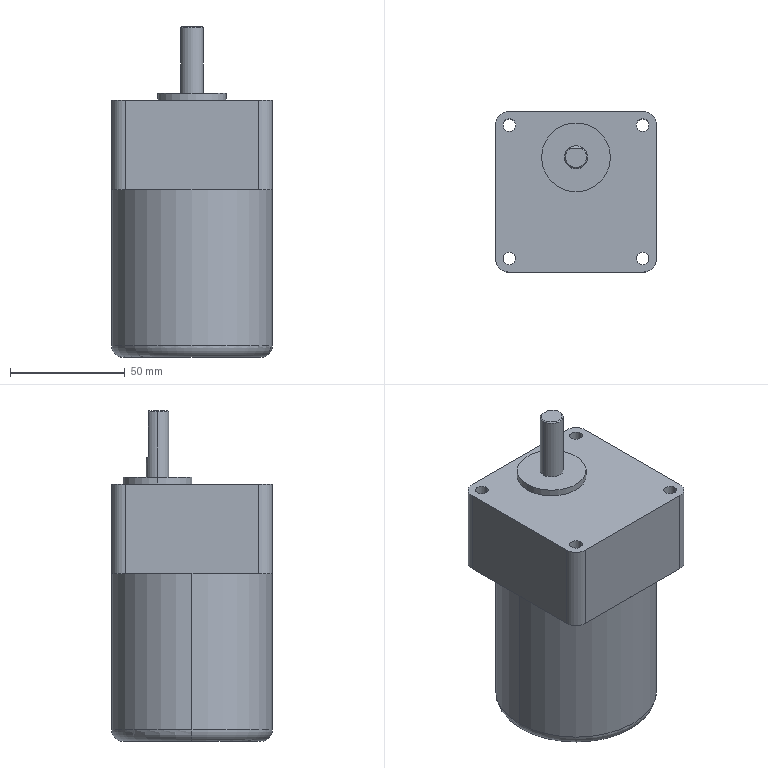Component | SolidWorks | LD101-02--Q1000-Q16-1.SLDQ1SM-1_LD101-02-3IK15Q1-C-3GN10K-1 | 1 solid | 37 faces | box 70 x 70 x 144 mm | volume 470295 mm3 | cylinder 18 | plane 14 | cone 3 | torus 2 | commonest cylinder face diameters 5.5 x8 12 x4 10 x2 30 x2 70 x2 | material SUS304
STEP:
#1=COLOUR_RGB('',0.7922,0.8196,0.9333);
#2=FILL_AREA_STYLE_COLOUR('',#1);
#3=FILL_AREA_STYLE('',(#2));
#4=SURFACE_STYLE_FILL_AREA(#3);
#5=SURFACE_SIDE_STYLE('',(#4));
#6=SURFACE_STYLE_USAGE(.BOTH.,#5);
#7=PRESENTATION_STYLE_ASSIGNMENT((#6));
#8=CARTESIAN_POINT('',(-28.624,-2.437,-4.714));
#9=VERTEX_POINT('',#8);
#10=CARTESIAN_POINT('',(-28.407,-2.437,-4.714));
#11=VERTEX_POINT('',#10);
#12=CARTESIAN_POINT('',(-28.516,-2.437,-4.714));
#13=DIRECTION('',(-0.,-0.,1.));
#14=DIRECTION('',(1.,0.,0.));
#15=AXIS2_PLACEMENT_3D('',#12,#13,#14);
#16=CIRCLE('',#15,0.1083);
#17=EDGE_CURVE('',#9,#11,#16,.T.);
#18=ORIENTED_EDGE('',*,*,#17,.F.);
#19=CARTESIAN_POINT('',(-28.624,-2.437,-3.179));
#20=VERTEX_POINT('',#19);
#21=CARTESIAN_POINT('',(-28.624,-2.437,-3.179));
#22=DIRECTION('',(-0.,-0.,1.));
#23=VECTOR('',#22,39.37);
#24=LINE('',#21,#23);
#25=EDGE_CURVE('',#9,#20,#24,.T.);
#26=ORIENTED_EDGE('',*,*,#25,.T.);
#27=CARTESIAN_POINT('',(-28.407,-2.437,-3.179));
#28=VERTEX_POINT('',#27);
#29=CARTESIAN_POINT('',(-28.516,-2.437,-3.179));
#30=DIRECTION('',(-0.,-0.,1.));
#31=DIRECTION('',(1.,0.,0.));
#32=AXIS2_PLACEMENT_3D('',#29,#30,#31);
#33=CIRCLE('',#32,0.1083);
#34=EDGE_CURVE('',#20,#28,#33,.T.);
#35=ORIENTED_EDGE('',*,*,#34,.T.);
#36=CARTESIAN_POINT('',(-28.407,-2.437,-3.179));
#37=DIRECTION('',(-0.,-0.,1.));
#38=VECTOR('',#37,39.37);
#39=LINE('',#36,#38);
#40=EDGE_CURVE('',#11,#28,#39,.T.);
#41=ORIENTED_EDGE('',*,*,#40,.F.);
#42=EDGE_LOOP('',(#18,#26,#35,#41));
#43=FACE_OUTER_BOUND('',#42,.T.);
#44=CARTESIAN_POINT('',(-28.516,-2.437,-3.179));
#45=DIRECTION('',(-0.,-0.,1.));
#46=DIRECTION('',(1.,0.,0.));
#47=AXIS2_PLACEMENT_3D('',#44,#45,#46);
#48=CYLINDRICAL_SURFACE('',#47,0.1083);
#49=ADVANCED_FACE('',(#43),#48,.F.);
#50=CARTESIAN_POINT('',(-28.624,-4.72,-4.714));
#51=VERTEX_POINT('',#50);
#52=CARTESIAN_POINT('',(-28.407,-4.72,-4.714));
#53=VERTEX_POINT('',#52);
#54=CARTESIAN_POINT('',(-28.516,-4.72,-4.714));
#55=DIRECTION('',(-0.,-0.,1.));
#56=DIRECTION('',(1.,0.,0.));
#57=AXIS2_PLACEMENT_3D('',#54,#55,#56);
#58=CIRCLE('',#57,0.1083);
#59=EDGE_CURVE('',#51,#53,#58,.T.);
#60=ORIENTED_EDGE('',*,*,#59,.F.);
#61=CARTESIAN_POINT('',(-28.624,-4.72,-3.179));
#62=VERTEX_POINT('',#61);
#63=CARTESIAN_POINT('',(-28.624,-4.72,-3.179));
#64=DIRECTION('',(-0.,-0.,1.));
#65=VECTOR('',#64,39.37);
#66=LINE('',#63,#65);
#67=EDGE_CURVE('',#51,#62,#66,.T.);
#68=ORIENTED_EDGE('',*,*,#67,.T.);
#69=CARTESIAN_POINT('',(-28.407,-4.72,-3.179));
#70=VERTEX_POINT('',#69);
#71=CARTESIAN_POINT('',(-28.516,-4.72,-3.179));
#72=DIRECTION('',(-0.,-0.,1.));
#73=DIRECTION('',(1.,0.,0.));
#74=AXIS2_PLACEMENT_3D('',#71,#72,#73);
#75=CIRCLE('',#74,0.1083);
#76=EDGE_CURVE('',#62,#70,#75,.T.);
#77=ORIENTED_EDGE('',*,*,#76,.T.);
#78=CARTESIAN_POINT('',(-28.407,-4.72,-3.179));
#79=DIRECTION('',(-0.,-0.,1.));
#80=VECTOR('',#79,39.37);
#81=LINE('',#78,#80);
#82=EDGE_CURVE('',#53,#70,#81,.T.);
#83=ORIENTED_EDGE('',*,*,#82,.F.);
#84=EDGE_LOOP('',(#60,#68,#77,#83));
#85=FACE_OUTER_BOUND('',#84,.T.);
#86=CARTESIAN_POINT('',(-28.516,-4.72,-3.179));
#87=DIRECTION('',(-0.,-0.,1.));
#88=DIRECTION('',(1.,0.,0.));
#89=AXIS2_PLACEMENT_3D('',#86,#87,#88);
#90=CYLINDRICAL_SURFACE('',#89,0.1083);
#91=ADVANCED_FACE('',(#85),#90,.F.);
#92=CARTESIAN_POINT('',(-30.907,-4.72,-4.714));
#93=VERTEX_POINT('',#92);
#94=CARTESIAN_POINT('',(-30.69,-4.72,-4.714));
#95=VERTEX_POINT('',#94);
#96=CARTESIAN_POINT('',(-30.798,-4.72,-4.714));
#97=DIRECTION('',(-0.,-0.,1.));
#98=DIRECTION('',(1.,0.,0.));
#99=AXIS2_PLACEMENT_3D('',#96,#97,#98);
#100=CIRCLE('',#99,0.1083);
#101=EDGE_CURVE('',#93,#95,#100,.T.);
#102=ORIENTED_EDGE('',*,*,#101,.F.);
#103=CARTESIAN_POINT('',(-30.907,-4.72,-3.179));
#104=VERTEX_POINT('',#103);
#105=CARTESIAN_POINT('',(-30.907,-4.72,-3.179));
#106=DIRECTION('',(-0.,-0.,1.));
#107=VECTOR('',#106,39.37);
#108=LINE('',#105,#107);
#109=EDGE_CURVE('',#93,#104,#108,.T.);
#110=ORIENTED_EDGE('',*,*,#109,.T.);
#111=CARTESIAN_POINT('',(-30.69,-4.72,-3.179));
#112=VERTEX_POINT('',#111);
#113=CARTESIAN_POINT('',(-30.798,-4.72,-3.179));
#114=DIRECTION('',(-0.,-0.,1.));
#115=DIRECTION('',(1.,0.,0.));
#116=AXIS2_PLACEMENT_3D('',#113,#114,#115);
#117=CIRCLE('',#116,0.1083);
#118=EDGE_CURVE('',#104,#112,#117,.T.);
#119=ORIENTED_EDGE('',*,*,#118,.T.);
#120=CARTESIAN_POINT('',(-30.69,-4.72,-3.179));
#121=DIRECTION('',(-0.,-0.,1.));
#122=VECTOR('',#121,39.37);
#123=LINE('',#120,#122);
#124=EDGE_CURVE('',#95,#112,#123,.T.);
#125=ORIENTED_EDGE('',*,*,#124,.F.);
#126=EDGE_LOOP('',(#102,#110,#119,#125));
#127=FACE_OUTER_BOUND('',#126,.T.);
#128=CARTESIAN_POINT('',(-30.798,-4.72,-3.179));
#129=DIRECTION('',(-0.,-0.,1.));
#130=DIRECTION('',(1.,0.,0.));
#131=AXIS2_PLACEMENT_3D('',#128,#129,#130);
#132=CYLINDRICAL_SURFACE('',#131,0.1083);
#133=ADVANCED_FACE('',(#127),#132,.F.);
#134=CARTESIAN_POINT('',(-30.907,-2.437,-4.714));
#135=VERTEX_POINT('',#134);
#136=CARTESIAN_POINT('',(-30.69,-2.437,-4.714));
#137=VERTEX_POINT('',#136);
#138=CARTESIAN_POINT('',(-30.798,-2.437,-4.714));
#139=DIRECTION('',(-0.,-0.,1.));
#140=DIRECTION('',(1.,0.,0.));
#141=AXIS2_PLACEMENT_3D('',#138,#139,#140);
#142=CIRCLE('',#141,0.1083);
#143=EDGE_CURVE('',#135,#137,#142,.T.);
#144=ORIENTED_EDGE('',*,*,#143,.F.);
#145=CARTESIAN_POINT('',(-30.907,-2.437,-3.179));
#146=VERTEX_POINT('',#145);
#147=CARTESIAN_POINT('',(-30.907,-2.437,-3.179));
#148=DIRECTION('',(-0.,-0.,1.));
#149=VECTOR('',#148,39.37);
#150=LINE('',#147,#149);
#151=EDGE_CURVE('',#135,#146,#150,.T.);
#152=ORIENTED_EDGE('',*,*,#151,.T.);
#153=CARTESIAN_POINT('',(-30.69,-2.437,-3.179));
#154=VERTEX_POINT('',#153);
#155=CARTESIAN_POINT('',(-30.798,-2.437,-3.179));
#156=DIRECTION('',(-0.,-0.,1.));
#157=DIRECTION('',(1.,0.,0.));
#158=AXIS2_PLACEMENT_3D('',#155,#156,#157);
#159=CIRCLE('',#158,0.1083);
#160=EDGE_CURVE('',#146,#154,#159,.T.);
#161=ORIENTED_EDGE('',*,*,#160,.T.);
#162=CARTESIAN_POINT('',(-30.69,-2.437,-3.179));
#163=DIRECTION('',(-0.,-0.,1.));
#164=VECTOR('',#163,39.37);
#165=LINE('',#162,#164);
#166=EDGE_CURVE('',#137,#154,#165,.T.);
#167=ORIENTED_EDGE('',*,*,#166,.F.);
#168=EDGE_LOOP('',(#144,#152,#161,#167));
#169=FACE_OUTER_BOUND('',#168,.T.);
#170=CARTESIAN_POINT('',(-30.798,-2.437,-3.179));
#171=DIRECTION('',(-0.,-0.,1.));
#172=DIRECTION('',(1.,0.,0.));
#173=AXIS2_PLACEMENT_3D('',#170,#171,#172);
#174=CYLINDRICAL_SURFACE('',#173,0.1083);
#175=ADVANCED_FACE('',(#169),#174,.F.);
#176=CARTESIAN_POINT('',(-29.48,-2.988,-1.919));
#177=VERTEX_POINT('',#176);
#178=CARTESIAN_POINT('',(-29.576,-2.831,-1.919));
#179=VERTEX_POINT('',#178);
#180=CARTESIAN_POINT('',(-29.657,-2.988,-1.919));
#181=DIRECTION('',(-0.,-0.,1.));
#182=DIRECTION('',(1.,0.,0.));
#183=AXIS2_PLACEMENT_3D('',#180,#181,#182);
#184=CIRCLE('',#183,0.1772);
#185=EDGE_CURVE('',#177,#179,#184,.T.);
#186=ORIENTED_EDGE('',*,*,#185,.F.);
#187=CARTESIAN_POINT('',(-29.46,-2.988,-1.939));
#188=VERTEX_POINT('',#187);
#189=CARTESIAN_POINT('',(-29.48,-2.988,-1.919));
#190=DIRECTION('',(0.7071,0.,-0.7071));
#191=VECTOR('',#190,39.37);
#192=LINE('',#189,#191);
#193=EDGE_CURVE('',#177,#188,#192,.T.);
#194=ORIENTED_EDGE('',*,*,#193,.T.);
#195=CARTESIAN_POINT('',(-29.539,-2.831,-1.939));
#196=VERTEX_POINT('',#195);
#197=CARTESIAN_POINT('',(-29.657,-2.988,-1.939));
#198=DIRECTION('',(0.,0.,-1.));
#199=DIRECTION('',(1.,0.,0.));
#200=AXIS2_PLACEMENT_3D('',#197,#198,#199);
#201=CIRCLE('',#200,0.1969);
#202=EDGE_CURVE('',#196,#188,#201,.T.);
#203=ORIENTED_EDGE('',*,*,#202,.F.);
#204=CARTESIAN_POINT('',(-29.576,-2.831,-1.919));
#205=CARTESIAN_POINT('',(-29.563,-2.831,-1.925));
#206=CARTESIAN_POINT('',(-29.551,-2.831,-1.932));
#207=CARTESIAN_POINT('',(-29.539,-2.831,-1.939));
#208=B_SPLINE_CURVE_WITH_KNOTS('',3,(#204,#205,#206,#207),.UNSPECIFIED.,.F.,.F.,(4,4),(0.01478,0.01585),.UNSPECIFIED.);
#209=EDGE_CURVE('',#179,#196,#208,.T.);
#210=ORIENTED_EDGE('',*,*,#209,.F.);
#211=EDGE_LOOP('',(#186,#194,#203,#210));
#212=FACE_OUTER_BOUND('',#211,.T.);
#213=CARTESIAN_POINT('',(-29.657,-2.988,-1.919));
#214=DIRECTION('',(0.,0.,-1.));
#215=DIRECTION('',(-1.,0.,0.));
#216=AXIS2_PLACEMENT_3D('',#213,#214,#215);
#217=CONICAL_SURFACE('',#216,0.1772,0.7854);
#218=ADVANCED_FACE('',(#212),#217,.T.);
#219=ORIENTED_EDGE('',*,*,#193,.F.);
#220=CARTESIAN_POINT('',(-29.834,-2.988,-1.919));
#221=VERTEX_POINT('',#220);
#222=CARTESIAN_POINT('',(-29.657,-2.988,-1.919));
#223=DIRECTION('',(-0.,-0.,1.));
#224=DIRECTION('',(1.,0.,0.));
#225=AXIS2_PLACEMENT_3D('',#222,#223,#224);
#226=CIRCLE('',#225,0.1772);
#227=EDGE_CURVE('',#221,#177,#226,.T.);
#228=ORIENTED_EDGE('',*,*,#227,.F.);
#229=CARTESIAN_POINT('',(-29.854,-2.988,-1.939));
#230=VERTEX_POINT('',#229);
#231=CARTESIAN_POINT('',(-29.834,-2.988,-1.919));
#232=DIRECTION('',(-0.7071,0.,-0.7071));
#233=VECTOR('',#232,39.37);
#234=LINE('',#231,#233);
#235=EDGE_CURVE('',#221,#230,#234,.T.);
#236=ORIENTED_EDGE('',*,*,#235,.T.);
#237=CARTESIAN_POINT('',(-29.657,-2.988,-1.939));
#238=DIRECTION('',(0.,0.,-1.));
#239=DIRECTION('',(1.,0.,0.));
#240=AXIS2_PLACEMENT_3D('',#237,#238,#239);
#241=CIRCLE('',#240,0.1969);
#242=EDGE_CURVE('',#188,#230,#241,.T.);
#243=ORIENTED_EDGE('',*,*,#242,.F.);
#244=EDGE_LOOP('',(#219,#228,#236,#243));
#245=FACE_OUTER_BOUND('',#244,.T.);
#246=CARTESIAN_POINT('',(-29.657,-2.988,-1.919));
#247=DIRECTION('',(0.,0.,-1.));
#248=DIRECTION('',(-1.,0.,0.));
#249=AXIS2_PLACEMENT_3D('',#246,#247,#248);
#250=CONICAL_SURFACE('',#249,0.1772,0.7854);
#251=ADVANCED_FACE('',(#245),#250,.T.);
#252=ORIENTED_EDGE('',*,*,#202,.T.);
#253=CARTESIAN_POINT('',(-29.46,-2.988,-3.061));
#254=VERTEX_POINT('',#253);
#255=CARTESIAN_POINT('',(-29.46,-2.988,-1.919));
#256=DIRECTION('',(0.,0.,-1.));
#257=VECTOR('',#256,39.37);
#258=LINE('',#255,#257);
#259=EDGE_CURVE('',#188,#254,#258,.T.);
#260=ORIENTED_EDGE('',*,*,#259,.T.);
#261=CARTESIAN_POINT('',(-29.854,-2.988,-3.061));
#262=VERTEX_POINT('',#261);
#263=CARTESIAN_POINT('',(-29.657,-2.988,-3.061));
#264=DIRECTION('',(0.,0.,-1.));
#265=DIRECTION('',(1.,0.,0.));
#266=AXIS2_PLACEMENT_3D('',#263,#264,#265);
#267=CIRCLE('',#266,0.1969);
#268=EDGE_CURVE('',#262,#254,#267,.T.);
#269=ORIENTED_EDGE('',*,*,#268,.F.);
#270=CARTESIAN_POINT('',(-29.854,-2.988,-1.919));
#271=DIRECTION('',(0.,0.,-1.));
#272=VECTOR('',#271,39.37);
#273=LINE('',#270,#272);
#274=EDGE_CURVE('',#230,#262,#273,.T.);
#275=ORIENTED_EDGE('',*,*,#274,.F.);
#276=CARTESIAN_POINT('',(-29.775,-2.831,-1.939));
#277=VERTEX_POINT('',#276);
#278=CARTESIAN_POINT('',(-29.657,-2.988,-1.939));
#279=DIRECTION('',(0.,0.,-1.));
#280=DIRECTION('',(1.,-0.,0.));
#281=AXIS2_PLACEMENT_3D('',#278,#279,#280);
#282=CIRCLE('',#281,0.1969);
#283=EDGE_CURVE('',#230,#277,#282,.T.);
#284=ORIENTED_EDGE('',*,*,#283,.T.);
#285=CARTESIAN_POINT('',(-29.775,-2.831,-2.706));
#286=VERTEX_POINT('',#285);
#287=CARTESIAN_POINT('',(-29.775,-2.831,-1.919));
#288=DIRECTION('',(0.,0.,-1.));
#289=VECTOR('',#288,39.37);
#290=LINE('',#287,#289);
#291=EDGE_CURVE('',#277,#286,#290,.T.);
#292=ORIENTED_EDGE('',*,*,#291,.T.);
#293=CARTESIAN_POINT('',(-29.539,-2.831,-2.706));
#294=VERTEX_POINT('',#293);
#295=CARTESIAN_POINT('',(-29.775,-2.831,-2.706));
#296=CARTESIAN_POINT('',(-29.703,-2.776,-2.761));
#297=CARTESIAN_POINT('',(-29.612,-2.776,-2.761));
#298=CARTESIAN_POINT('',(-29.539,-2.831,-2.706));
#299=(BOUNDED_CURVE()B_SPLINE_CURVE(3,(#295,#296,#297,#298),.UNSPECIFIED.,.F.,.F.)B_SPLINE_CURVE_WITH_KNOTS((4,4),(5.64,6.927),.UNSPECIFIED.)CURVE()GEOMETRIC_REPRESENTATION_ITEM()RATIONAL_B_SPLINE_CURVE((1.,0.8667,0.8667,1.))REPRESENTATION_ITEM(''));
#300=EDGE_CURVE('',#286,#294,#299,.T.);
#301=ORIENTED_EDGE('',*,*,#300,.T.);
#302=CARTESIAN_POINT('',(-29.539,-2.831,-1.919));
#303=DIRECTION('',(-0.,-0.,1.));
#304=VECTOR('',#303,39.37);
#305=LINE('',#302,#304);
#306=EDGE_CURVE('',#294,#196,#305,.T.);
#307=ORIENTED_EDGE('',*,*,#306,.T.);
#308=EDGE_LOOP('',(#252,#260,#269,#275,#284,#292,#301,#307));
#309=FACE_OUTER_BOUND('',#308,.T.);
#310=CARTESIAN_POINT('',(-29.657,-2.988,-1.919));
#311=DIRECTION('',(0.,0.,-1.));
#312=DIRECTION('',(-1.,0.,0.));
#313=AXIS2_PLACEMENT_3D('',#310,#311,#312);
#314=CYLINDRICAL_SURFACE('',#313,0.1969);
#315=ADVANCED_FACE('',(#309),#314,.T.);
#316=CARTESIAN_POINT('',(-29.067,-2.988,-3.061));
#317=VERTEX_POINT('',#316);
#318=CARTESIAN_POINT('',(-30.248,-2.988,-3.061));
#319=VERTEX_POINT('',#318);
#320=CARTESIAN_POINT('',(-29.657,-2.988,-3.061));
#321=DIRECTION('',(-0.,-0.,1.));
#322=DIRECTION('',(1.,0.,0.));
#323=AXIS2_PLACEMENT_3D('',#320,#321,#322);
#324=CIRCLE('',#323,0.5906);
#325=EDGE_CURVE('',#317,#319,#324,.T.);
#326=ORIENTED_EDGE('',*,*,#325,.F.);
#327=CARTESIAN_POINT('',(-29.067,-2.988,-3.179));
#328=VERTEX_POINT('',#327);
#329=CARTESIAN_POINT('',(-29.067,-2.988,-3.061));
#330=DIRECTION('',(0.,0.,-1.));
#331=VECTOR('',#330,39.37);
#332=LINE('',#329,#331);
#333=EDGE_CURVE('',#317,#328,#332,.T.);
#334=ORIENTED_EDGE('',*,*,#333,.T.);
#335=CARTESIAN_POINT('',(-30.248,-2.988,-3.179));
#336=VERTEX_POINT('',#335);
#337=CARTESIAN_POINT('',(-29.657,-2.988,-3.179));
#338=DIRECTION('',(-0.,-0.,1.));
#339=DIRECTION('',(1.,0.,0.));
#340=AXIS2_PLACEMENT_3D('',#337,#338,#339);
#341=CIRCLE('',#340,0.5906);
#342=EDGE_CURVE('',#328,#336,#341,.T.);
#343=ORIENTED_EDGE('',*,*,#342,.T.);
#344=CARTESIAN_POINT('',(-30.248,-2.988,-3.061));
#345=DIRECTION('',(0.,0.,-1.));
#346=VECTOR('',#345,39.37);
#347=LINE('',#344,#346);
#348=EDGE_CURVE('',#319,#336,#347,.T.);
#349=ORIENTED_EDGE('',*,*,#348,.F.);
#350=EDGE_LOOP('',(#326,#334,#343,#349));
#351=FACE_OUTER_BOUND('',#350,.T.);
#352=CARTESIAN_POINT('',(-29.657,-2.988,-3.061));
#353=DIRECTION('',(0.,0.,-1.));
#354=DIRECTION('',(-1.,0.,-0.));
#355=AXIS2_PLACEMENT_3D('',#352,#353,#354);
#356=CYLINDRICAL_SURFACE('',#355,0.5906);
#357=ADVANCED_FACE('',(#351),#356,.T.);
#358=CARTESIAN_POINT('',(-30.838,-3.579,-7.588));
#359=VERTEX_POINT('',#358);
#360=CARTESIAN_POINT('',(-28.476,-3.579,-7.588));
#361=VERTEX_POINT('',#360);
#362=CARTESIAN_POINT('',(-29.657,-3.579,-7.588));
#363=DIRECTION('',(0.,0.,-1.));
#364=DIRECTION('',(1.,0.,0.));
#365=AXIS2_PLACEMENT_3D('',#362,#363,#364);
#366=CIRCLE('',#365,1.181);
#367=EDGE_CURVE('',#359,#361,#366,.T.);
#368=ORIENTED_EDGE('',*,*,#367,.F.);
#369=CARTESIAN_POINT('',(-31.035,-3.579,-7.391));
#370=VERTEX_POINT('',#369);
#371=CARTESIAN_POINT('',(-30.838,-3.579,-7.391));
#372=DIRECTION('',(0.,1.,0.));
#373=DIRECTION('',(-1.,0.,0.));
#374=AXIS2_PLACEMENT_3D('',#371,#372,#373);
#375=CIRCLE('',#374,0.1969);
#376=EDGE_CURVE('',#359,#370,#375,.T.);
#377=ORIENTED_EDGE('',*,*,#376,.T.);
#378=CARTESIAN_POINT('',(-28.279,-3.579,-7.391));
#379=VERTEX_POINT('',#378);
#380=CARTESIAN_POINT('',(-29.657,-3.579,-7.391));
#381=DIRECTION('',(-0.,-0.,1.));
#382=DIRECTION('',(1.,0.,0.));
#383=AXIS2_PLACEMENT_3D('',#380,#381,#382);
#384=CIRCLE('',#383,1.378);
#385=EDGE_CURVE('',#379,#370,#384,.T.);
#386=ORIENTED_EDGE('',*,*,#385,.F.);
#387=CARTESIAN_POINT('',(-28.476,-3.579,-7.391));
#388=DIRECTION('',(-0.,-1.,-0.));
#389=DIRECTION('',(1.,0.,0.));
#390=AXIS2_PLACEMENT_3D('',#387,#388,#389);
#391=CIRCLE('',#390,0.1969);
#392=EDGE_CURVE('',#361,#379,#391,.T.);
#393=ORIENTED_EDGE('',*,*,#392,.F.);
#394=EDGE_LOOP('',(#368,#377,#386,#393));
#395=FACE_OUTER_BOUND('',#394,.T.);
#396=CARTESIAN_POINT('',(-29.657,-3.579,-7.391));
#397=DIRECTION('',(-0.,-0.,1.));
#398=DIRECTION('',(1.,0.,0.));
#399=AXIS2_PLACEMENT_3D('',#396,#397,#398);
#400=TOROIDAL_SURFACE('',#399,1.181,0.1969);
#401=ADVANCED_FACE('',(#395),#400,.T.);
#402=ORIENTED_EDGE('',*,*,#385,.T.);
#403=CARTESIAN_POINT('',(-31.035,-3.579,-4.714));
#404=VERTEX_POINT('',#403);
#405=CARTESIAN_POINT('',(-31.035,-3.579,-7.588));
#406=DIRECTION('',(-0.,-0.,1.));
#407=VECTOR('',#406,39.37);
#408=LINE('',#405,#407);
#409=EDGE_CURVE('',#370,#404,#408,.T.);
#410=ORIENTED_EDGE('',*,*,#409,.T.);
#411=CARTESIAN_POINT('',(-29.657,-2.201,-4.714));
#412=VERTEX_POINT('',#411);
#413=CARTESIAN_POINT('',(-29.657,-3.579,-4.714));
#414=DIRECTION('',(-0.,-0.,1.));
#415=DIRECTION('',(1.,0.,0.));
#416=AXIS2_PLACEMENT_3D('',#413,#414,#415);
#417=CIRCLE('',#416,1.378);
#418=EDGE_CURVE('',#412,#404,#417,.T.);
#419=ORIENTED_EDGE('',*,*,#418,.F.);
#420=CARTESIAN_POINT('',(-28.279,-3.579,-4.714));
#421=VERTEX_POINT('',#420);
#422=CARTESIAN_POINT('',(-29.657,-3.579,-4.714));
#423=DIRECTION('',(-0.,-0.,1.));
#424=DIRECTION('',(1.,0.,0.));
#425=AXIS2_PLACEMENT_3D('',#422,#423,#424);
#426=CIRCLE('',#425,1.378);
#427=EDGE_CURVE('',#421,#412,#426,.T.);
#428=ORIENTED_EDGE('',*,*,#427,.F.);
#429=CARTESIAN_POINT('',(-28.279,-3.579,-7.588));
#430=DIRECTION('',(-0.,-0.,1.));
#431=VECTOR('',#430,39.37);
#432=LINE('',#429,#431);
#433=EDGE_CURVE('',#379,#421,#432,.T.);
#434=ORIENTED_EDGE('',*,*,#433,.F.);
#435=EDGE_LOOP('',(#402,#410,#419,#428,#434));
#436=FACE_OUTER_BOUND('',#435,.T.);
#437=CARTESIAN_POINT('',(-29.657,-3.579,-7.588));
#438=DIRECTION('',(-0.,-0.,1.));
#439=DIRECTION('',(1.,0.,0.));
#440=AXIS2_PLACEMENT_3D('',#437,#438,#439);
#441=CYLINDRICAL_SURFACE('',#440,1.378);
#442=ADVANCED_FACE('',(#436),#441,.T.);
#443=CARTESIAN_POINT('',(-29.657,-2.988,-3.061));
#444=DIRECTION('',(-0.,-0.,1.));
#445=DIRECTION('',(1.,0.,0.));
#446=AXIS2_PLACEMENT_3D('',#443,#444,#445);
#447=CIRCLE('',#446,0.5906);
#448=EDGE_CURVE('',#319,#317,#447,.T.);
#449=ORIENTED_EDGE('',*,*,#448,.T.);
#450=ORIENTED_EDGE('',*,*,#325,.T.);
#451=EDGE_LOOP('',(#449,#450));
#452=FACE_OUTER_BOUND('',#451,.T.);
#453=ORIENTED_EDGE('',*,*,#268,.T.);
#454=CARTESIAN_POINT('',(-29.657,-2.988,-3.061));
#455=DIRECTION('',(0.,0.,-1.));
#456=DIRECTION('',(1.,0.,0.));
#457=AXIS2_PLACEMENT_3D('',#454,#455,#456);
#458=CIRCLE('',#457,0.1969);
#459=EDGE_CURVE('',#254,#262,#458,.T.);
#460=ORIENTED_EDGE('',*,*,#459,.T.);
#461=EDGE_LOOP('',(#453,#460));
#462=FACE_BOUND('',#461,.T.);
#463=CARTESIAN_POINT('',(-29.657,-2.988,-3.061));
#464=DIRECTION('',(-0.,-0.,1.));
#465=DIRECTION('',(1.,-0.,0.));
#466=AXIS2_PLACEMENT_3D('',#463,#464,#465);
#467=PLANE('',#466);
#468=ADVANCED_FACE('',(#452,#462),#467,.T.);
#469=CARTESIAN_POINT('',(-28.516,-2.437,-3.179));
#470=DIRECTION('',(-0.,-0.,1.));
#471=DIRECTION('',(1.,0.,0.));
#472=AXIS2_PLACEMENT_3D('',#469,#470,#471);
#473=CIRCLE('',#472,0.1083);
#474=EDGE_CURVE('',#28,#20,#473,.T.);
#475=ORIENTED_EDGE('',*,*,#474,.F.);
#476=ORIENTED_EDGE('',*,*,#34,.F.);
#477=EDGE_LOOP('',(#475,#476));
#478=FACE_BOUND('',#477,.T.);
#479=CARTESIAN_POINT('',(-28.516,-4.72,-3.179));
#480=DIRECTION('',(-0.,-0.,1.));
#481=DIRECTION('',(1.,0.,0.));
#482=AXIS2_PLACEMENT_3D('',#479,#480,#481);
#483=CIRCLE('',#482,0.1083);
#484=EDGE_CURVE('',#70,#62,#483,.T.);
#485=ORIENTED_EDGE('',*,*,#484,.F.);
#486=ORIENTED_EDGE('',*,*,#76,.F.);
#487=EDGE_LOOP('',(#485,#486));
#488=FACE_BOUND('',#487,.T.);
#489=CARTESIAN_POINT('',(-30.798,-4.72,-3.179));
#490=DIRECTION('',(-0.,-0.,1.));
#491=DIRECTION('',(1.,0.,0.));
#492=AXIS2_PLACEMENT_3D('',#489,#490,#491);
#493=CIRCLE('',#492,0.1083);
#494=EDGE_CURVE('',#112,#104,#493,.T.);
#495=ORIENTED_EDGE('',*,*,#494,.F.);
#496=ORIENTED_EDGE('',*,*,#118,.F.);
#497=EDGE_LOOP('',(#495,#496));
#498=FACE_BOUND('',#497,.T.);
#499=CARTESIAN_POINT('',(-30.798,-2.437,-3.179));
#500=DIRECTION('',(-0.,-0.,1.));
#501=DIRECTION('',(1.,0.,0.));
#502=AXIS2_PLACEMENT_3D('',#499,#500,#501);
#503=CIRCLE('',#502,0.1083);
#504=EDGE_CURVE('',#154,#146,#503,.T.);
#505=ORIENTED_EDGE('',*,*,#504,.F.);
#506=ORIENTED_EDGE('',*,*,#160,.F.);
#507=EDGE_LOOP('',(#505,#506));
#508=FACE_BOUND('',#507,.T.);
#509=CARTESIAN_POINT('',(-28.515,-4.957,-3.179));
#510=VERTEX_POINT('',#509);
#511=CARTESIAN_POINT('',(-28.279,-4.72,-3.179));
#512=VERTEX_POINT('',#511);
#513=CARTESIAN_POINT('',(-28.515,-4.72,-3.179));
#514=DIRECTION('',(-0.,-0.,1.));
#515=DIRECTION('',(1.,0.,0.));
#516=AXIS2_PLACEMENT_3D('',#513,#514,#515);
#517=CIRCLE('',#516,0.2362);
#518=EDGE_CURVE('',#510,#512,#517,.T.);
#519=ORIENTED_EDGE('',*,*,#518,.T.);
#520=CARTESIAN_POINT('',(-28.279,-2.437,-3.179));
#521=VERTEX_POINT('',#520);
#522=CARTESIAN_POINT('',(-28.279,-4.72,-3.179));
#523=DIRECTION('',(-0.,1.,0.));
#524=VECTOR('',#523,39.37);
#525=LINE('',#522,#524);
#526=EDGE_CURVE('',#512,#521,#525,.T.);
#527=ORIENTED_EDGE('',*,*,#526,.T.);
#528=CARTESIAN_POINT('',(-28.515,-2.201,-3.179));
#529=VERTEX_POINT('',#528);
#530=CARTESIAN_POINT('',(-28.515,-2.437,-3.179));
#531=DIRECTION('',(-0.,-0.,1.));
#532=DIRECTION('',(1.,0.,0.));
#533=AXIS2_PLACEMENT_3D('',#530,#531,#532);
#534=CIRCLE('',#533,0.2362);
#535=EDGE_CURVE('',#521,#529,#534,.T.);
#536=ORIENTED_EDGE('',*,*,#535,.T.);
#537=CARTESIAN_POINT('',(-30.799,-2.201,-3.179));
#538=VERTEX_POINT('',#537);
#539=CARTESIAN_POINT('',(-28.515,-2.201,-3.179));
#540=DIRECTION('',(-1.,0.,-0.));
#541=VECTOR('',#540,39.37);
#542=LINE('',#539,#541);
#543=EDGE_CURVE('',#529,#538,#542,.T.);
#544=ORIENTED_EDGE('',*,*,#543,.T.);
#545=CARTESIAN_POINT('',(-31.035,-2.437,-3.179));
#546=VERTEX_POINT('',#545);
#547=CARTESIAN_POINT('',(-30.799,-2.437,-3.179));
#548=DIRECTION('',(-0.,-0.,1.));
#549=DIRECTION('',(1.,0.,0.));
#550=AXIS2_PLACEMENT_3D('',#547,#548,#549);
#551=CIRCLE('',#550,0.2362);
#552=EDGE_CURVE('',#538,#546,#551,.T.);
#553=ORIENTED_EDGE('',*,*,#552,.T.);
#554=CARTESIAN_POINT('',(-31.035,-4.72,-3.179));
#555=VERTEX_POINT('',#554);
#556=CARTESIAN_POINT('',(-31.035,-2.437,-3.179));
#557=DIRECTION('',(-0.,-1.,-0.));
#558=VECTOR('',#557,39.37);
#559=LINE('',#556,#558);
#560=EDGE_CURVE('',#546,#555,#559,.T.);
#561=ORIENTED_EDGE('',*,*,#560,.T.);
#562=CARTESIAN_POINT('',(-30.799,-4.957,-3.179));
#563=VERTEX_POINT('',#562);
#564=CARTESIAN_POINT('',(-30.799,-4.72,-3.179));
#565=DIRECTION('',(-0.,-0.,1.));
#566=DIRECTION('',(1.,0.,0.));
#567=AXIS2_PLACEMENT_3D('',#564,#565,#566);
#568=CIRCLE('',#567,0.2362);
#569=EDGE_CURVE('',#555,#563,#568,.T.);
#570=ORIENTED_EDGE('',*,*,#569,.T.);
#571=CARTESIAN_POINT('',(-30.799,-4.957,-3.179));
#572=DIRECTION('',(1.,0.,0.));
#573=VECTOR('',#572,39.37);
#574=LINE('',#571,#573);
#575=EDGE_CURVE('',#563,#510,#574,.T.);
#576=ORIENTED_EDGE('',*,*,#575,.T.);
#577=EDGE_LOOP('',(#519,#527,#536,#544,#553,#561,#570,#576));
#578=FACE_OUTER_BOUND('',#577,.T.);
#579=CARTESIAN_POINT('',(-29.657,-2.988,-3.179));
#580=DIRECTION('',(-0.,-0.,1.));
#581=DIRECTION('',(1.,0.,0.));
#582=AXIS2_PLACEMENT_3D('',#579,#580,#581);
#583=CIRCLE('',#582,0.5906);
#584=EDGE_CURVE('',#336,#328,#583,.T.);
#585=ORIENTED_EDGE('',*,*,#584,.F.);
#586=ORIENTED_EDGE('',*,*,#342,.F.);
#587=EDGE_LOOP('',(#585,#586));
#588=FACE_BOUND('',#587,.T.);
#589=CARTESIAN_POINT('',(-28.515,-4.72,-3.179));
#590=DIRECTION('',(-0.,-0.,1.));
#591=DIRECTION('',(1.,-0.,0.));
#592=AXIS2_PLACEMENT_3D('',#589,#590,#591);
#593=PLANE('',#592);
#594=ADVANCED_FACE('',(#478,#488,#498,#508,#578,#588),#593,.T.);
#595=CARTESIAN_POINT('',(-28.516,-2.437,-4.714));
#596=DIRECTION('',(-0.,-0.,1.));
#597=DIRECTION('',(1.,0.,0.));
#598=AXIS2_PLACEMENT_3D('',#595,#596,#597);
#599=CIRCLE('',#598,0.1083);
#600=EDGE_CURVE('',#11,#9,#599,.T.);
#601=ORIENTED_EDGE('',*,*,#600,.T.);
#602=ORIENTED_EDGE('',*,*,#17,.T.);
#603=EDGE_LOOP('',(#601,#602));
#604=FACE_BOUND('',#603,.T.);
#605=CARTESIAN_POINT('',(-28.279,-2.437,-4.714));
#606=VERTEX_POINT('',#605);
#607=CARTESIAN_POINT('',(-28.279,-4.72,-4.714));
#608=DIRECTION('',(-0.,1.,0.));
#609=VECTOR('',#608,39.37);
#610=LINE('',#607,#609);
#611=EDGE_CURVE('',#421,#606,#610,.T.);
#612=ORIENTED_EDGE('',*,*,#611,.F.);
#613=ORIENTED_EDGE('',*,*,#427,.T.);
#614=CARTESIAN_POINT('',(-28.515,-2.201,-4.714));
#615=VERTEX_POINT('',#614);
#616=CARTESIAN_POINT('',(-30.799,-2.201,-4.714));
#617=DIRECTION('',(-1.,-0.,-0.));
#618=VECTOR('',#617,39.37);
#619=LINE('',#616,#618);
#620=EDGE_CURVE('',#615,#412,#619,.T.);
#621=ORIENTED_EDGE('',*,*,#620,.F.);
#622=CARTESIAN_POINT('',(-28.515,-2.437,-4.714));
#623=DIRECTION('',(-0.,-0.,1.));
#624=DIRECTION('',(1.,0.,0.));
#625=AXIS2_PLACEMENT_3D('',#622,#623,#624);
#626=CIRCLE('',#625,0.2362);
#627=EDGE_CURVE('',#606,#615,#626,.T.);
#628=ORIENTED_EDGE('',*,*,#627,.F.);
#629=EDGE_LOOP('',(#612,#613,#621,#628));
#630=FACE_OUTER_BOUND('',#629,.T.);
#631=CARTESIAN_POINT('',(-30.799,-4.72,-4.714));
#632=DIRECTION('',(-0.,-0.,1.));
#633=DIRECTION('',(1.,-0.,0.));
#634=AXIS2_PLACEMENT_3D('',#631,#632,#633);
#635=PLANE('',#634);
#636=ADVANCED_FACE('',(#604,#630),#635,.F.);
#637=CARTESIAN_POINT('',(-30.798,-2.437,-4.714));
#638=DIRECTION('',(-0.,-0.,1.));
#639=DIRECTION('',(1.,0.,0.));
#640=AXIS2_PLACEMENT_3D('',#637,#638,#639);
#641=CIRCLE('',#640,0.1083);
#642=EDGE_CURVE('',#137,#135,#641,.T.);
#643=ORIENTED_EDGE('',*,*,#642,.T.);
#644=ORIENTED_EDGE('',*,*,#143,.T.);
#645=EDGE_LOOP('',(#643,#644));
#646=FACE_BOUND('',#645,.T.);
#647=CARTESIAN_POINT('',(-30.799,-2.201,-4.714));
#648=VERTEX_POINT('',#647);
#649=CARTESIAN_POINT('',(-30.799,-2.201,-4.714));
#650=DIRECTION('',(-1.,-0.,-0.));
#651=VECTOR('',#650,39.37);
#652=LINE('',#649,#651);
#653=EDGE_CURVE('',#412,#648,#652,.T.);
#654=ORIENTED_EDGE('',*,*,#653,.F.);
#655=ORIENTED_EDGE('',*,*,#418,.T.);
#656=CARTESIAN_POINT('',(-31.035,-2.437,-4.714));
#657=VERTEX_POINT('',#656);
#658=CARTESIAN_POINT('',(-31.035,-4.72,-4.714));
#659=DIRECTION('',(-0.,-1.,-0.));
#660=VECTOR('',#659,39.37);
#661=LINE('',#658,#660);
#662=EDGE_CURVE('',#657,#404,#661,.T.);
#663=ORIENTED_EDGE('',*,*,#662,.F.);
#664=CARTESIAN_POINT('',(-30.799,-2.437,-4.714));
#665=DIRECTION('',(-0.,-0.,1.));
#666=DIRECTION('',(1.,0.,0.));
#667=AXIS2_PLACEMENT_3D('',#664,#665,#666);
#668=CIRCLE('',#667,0.2362);
#669=EDGE_CURVE('',#648,#657,#668,.T.);
#670=ORIENTED_EDGE('',*,*,#669,.F.);
#671=EDGE_LOOP('',(#654,#655,#663,#670));
#672=FACE_OUTER_BOUND('',#671,.T.);
#673=CARTESIAN_POINT('',(-30.799,-4.72,-4.714));
#674=DIRECTION('',(-0.,-0.,1.));
#675=DIRECTION('',(1.,-0.,0.));
#676=AXIS2_PLACEMENT_3D('',#673,#674,#675);
#677=PLANE('',#676);
#678=ADVANCED_FACE('',(#646,#672),#677,.F.);
#679=CARTESIAN_POINT('',(-30.798,-4.72,-4.714));
#680=DIRECTION('',(-0.,-0.,1.));
#681=DIRECTION('',(1.,0.,0.));
#682=AXIS2_PLACEMENT_3D('',#679,#680,#681);
#683=CIRCLE('',#682,0.1083);
#684=EDGE_CURVE('',#95,#93,#683,.T.);
#685=ORIENTED_EDGE('',*,*,#684,.T.);
#686=ORIENTED_EDGE('',*,*,#101,.T.);
#687=EDGE_LOOP('',(#685,#686));
#688=FACE_BOUND('',#687,.T.);
#689=CARTESIAN_POINT('',(-31.035,-4.72,-4.714));
#690=VERTEX_POINT('',#689);
#691=CARTESIAN_POINT('',(-31.035,-4.72,-4.714));
#692=DIRECTION('',(-0.,-1.,-0.));
#693=VECTOR('',#692,39.37);
#694=LINE('',#691,#693);
#695=EDGE_CURVE('',#404,#690,#694,.T.);
#696=ORIENTED_EDGE('',*,*,#695,.F.);
#697=CARTESIAN_POINT('',(-29.657,-4.957,-4.714));
#698=VERTEX_POINT('',#697);
#699=CARTESIAN_POINT('',(-29.657,-3.579,-4.714));
#700=DIRECTION('',(-0.,-0.,1.));
#701=DIRECTION('',(1.,0.,0.));
#702=AXIS2_PLACEMENT_3D('',#699,#700,#701);
#703=CIRCLE('',#702,1.378);
#704=EDGE_CURVE('',#404,#698,#703,.T.);
#705=ORIENTED_EDGE('',*,*,#704,.T.);
#706=CARTESIAN_POINT('',(-30.799,-4.957,-4.714));
#707=VERTEX_POINT('',#706);
#708=CARTESIAN_POINT('',(-30.799,-4.957,-4.714));
#709=DIRECTION('',(1.,0.,0.));
#710=VECTOR('',#709,39.37);
#711=LINE('',#708,#710);
#712=EDGE_CURVE('',#707,#698,#711,.T.);
#713=ORIENTED_EDGE('',*,*,#712,.F.);
#714=CARTESIAN_POINT('',(-30.799,-4.72,-4.714));
#715=DIRECTION('',(-0.,-0.,1.));
#716=DIRECTION('',(1.,0.,0.));
#717=AXIS2_PLACEMENT_3D('',#714,#715,#716);
#718=CIRCLE('',#717,0.2362);
#719=EDGE_CURVE('',#690,#707,#718,.T.);
#720=ORIENTED_EDGE('',*,*,#719,.F.);
#721=EDGE_LOOP('',(#696,#705,#713,#720));
#722=FACE_OUTER_BOUND('',#721,.T.);
#723=CARTESIAN_POINT('',(-30.799,-4.72,-4.714));
#724=DIRECTION('',(-0.,-0.,1.));
#725=DIRECTION('',(1.,-0.,0.));
#726=AXIS2_PLACEMENT_3D('',#723,#724,#725);
#727=PLANE('',#726);
#728=ADVANCED_FACE('',(#688,#722),#727,.F.);
#729=CARTESIAN_POINT('',(-30.799,-4.957,-4.714));
#730=DIRECTION('',(-0.,-0.,1.));
#731=VECTOR('',#730,39.37);
#732=LINE('',#729,#731);
#733=EDGE_CURVE('',#707,#563,#732,.T.);
#734=ORIENTED_EDGE('',*,*,#733,.T.);
#735=ORIENTED_EDGE('',*,*,#569,.F.);
#736=CARTESIAN_POINT('',(-31.035,-4.72,-4.714));
#737=DIRECTION('',(-0.,-0.,1.));
#738=VECTOR('',#737,39.37);
#739=LINE('',#736,#738);
#740=EDGE_CURVE('',#690,#555,#739,.T.);
#741=ORIENTED_EDGE('',*,*,#740,.F.);
#742=ORIENTED_EDGE('',*,*,#719,.T.);
#743=EDGE_LOOP('',(#734,#735,#741,#742));
#744=FACE_OUTER_BOUND('',#743,.T.);
#745=CARTESIAN_POINT('',(-30.799,-4.72,-4.714));
#746=DIRECTION('',(-0.,-0.,1.));
#747=DIRECTION('',(1.,0.,0.));
#748=AXIS2_PLACEMENT_3D('',#745,#746,#747);
#749=CYLINDRICAL_SURFACE('',#748,0.2362);
#750=ADVANCED_FACE('',(#744),#749,.T.);
#751=ORIENTED_EDGE('',*,*,#740,.T.);
#752=ORIENTED_EDGE('',*,*,#560,.F.);
#753=CARTESIAN_POINT('',(-31.035,-2.437,-4.714));
#754=DIRECTION('',(-0.,-0.,1.));
#755=VECTOR('',#754,39.37);
#756=LINE('',#753,#755);
#757=EDGE_CURVE('',#657,#546,#756,.T.);
#758=ORIENTED_EDGE('',*,*,#757,.F.);
#759=ORIENTED_EDGE('',*,*,#662,.T.);
#760=ORIENTED_EDGE('',*,*,#695,.T.);
#761=EDGE_LOOP('',(#751,#752,#758,#759,#760));
#762=FACE_OUTER_BOUND('',#761,.T.);
#763=CARTESIAN_POINT('',(-31.035,-4.72,-4.714));
#764=DIRECTION('',(-1.,0.,-0.));
#765=DIRECTION('',(-0.,-0.,1.));
#766=AXIS2_PLACEMENT_3D('',#763,#764,#765);
#767=PLANE('',#766);
#768=ADVANCED_FACE('',(#762),#767,.T.);
#769=ORIENTED_EDGE('',*,*,#757,.T.);
#770=ORIENTED_EDGE('',*,*,#552,.F.);
#771=CARTESIAN_POINT('',(-30.799,-2.201,-4.714));
#772=DIRECTION('',(-0.,-0.,1.));
#773=VECTOR('',#772,39.37);
#774=LINE('',#771,#773);
#775=EDGE_CURVE('',#648,#538,#774,.T.);
#776=ORIENTED_EDGE('',*,*,#775,.F.);
#777=ORIENTED_EDGE('',*,*,#669,.T.);
#778=EDGE_LOOP('',(#769,#770,#776,#777));
#779=FACE_OUTER_BOUND('',#778,.T.);
#780=CARTESIAN_POINT('',(-30.799,-2.437,-4.714));
#781=DIRECTION('',(-0.,-0.,1.));
#782=DIRECTION('',(1.,0.,0.));
#783=AXIS2_PLACEMENT_3D('',#780,#781,#782);
#784=CYLINDRICAL_SURFACE('',#783,0.2362);
#785=ADVANCED_FACE('',(#779),#784,.T.);
#786=ORIENTED_EDGE('',*,*,#775,.T.);
#787=ORIENTED_EDGE('',*,*,#543,.F.);
#788=CARTESIAN_POINT('',(-28.515,-2.201,-4.714));
#789=DIRECTION('',(-0.,-0.,1.));
#790=VECTOR('',#789,39.37);
#791=LINE('',#788,#790);
#792=EDGE_CURVE('',#615,#529,#791,.T.);
#793=ORIENTED_EDGE('',*,*,#792,.F.);
#794=ORIENTED_EDGE('',*,*,#620,.T.);
#795=ORIENTED_EDGE('',*,*,#653,.T.);
#796=EDGE_LOOP('',(#786,#787,#793,#794,#795));
#797=FACE_OUTER_BOUND('',#796,.T.);
#798=CARTESIAN_POINT('',(-30.799,-2.201,-4.714));
#799=DIRECTION('',(-0.,1.,0.));
#800=DIRECTION('',(-1.,-0.,-0.));
#801=AXIS2_PLACEMENT_3D('',#798,#799,#800);
#802=PLANE('',#801);
#803=ADVANCED_FACE('',(#797),#802,.T.);
#804=ORIENTED_EDGE('',*,*,#792,.T.);
#805=ORIENTED_EDGE('',*,*,#535,.F.);
#806=CARTESIAN_POINT('',(-28.279,-2.437,-4.714));
#807=DIRECTION('',(-0.,-0.,1.));
#808=VECTOR('',#807,39.37);
#809=LINE('',#806,#808);
#810=EDGE_CURVE('',#606,#521,#809,.T.);
#811=ORIENTED_EDGE('',*,*,#810,.F.);
#812=ORIENTED_EDGE('',*,*,#627,.T.);
#813=EDGE_LOOP('',(#804,#805,#811,#812));
#814=FACE_OUTER_BOUND('',#813,.T.);
#815=CARTESIAN_POINT('',(-28.515,-2.437,-4.714));
#816=DIRECTION('',(-0.,-0.,1.));
#817=DIRECTION('',(1.,0.,0.));
#818=AXIS2_PLACEMENT_3D('',#815,#816,#817);
#819=CYLINDRICAL_SURFACE('',#818,0.2362);
#820=ADVANCED_FACE('',(#814),#819,.T.);
#821=ORIENTED_EDGE('',*,*,#810,.T.);
#822=ORIENTED_EDGE('',*,*,#526,.F.);
#823=CARTESIAN_POINT('',(-28.279,-4.72,-4.714));
#824=VERTEX_POINT('',#823);
#825=CARTESIAN_POINT('',(-28.279,-4.72,-4.714));
#826=DIRECTION('',(-0.,-0.,1.));
#827=VECTOR('',#826,39.37);
#828=LINE('',#825,#827);
#829=EDGE_CURVE('',#824,#512,#828,.T.);
#830=ORIENTED_EDGE('',*,*,#829,.F.);
#831=CARTESIAN_POINT('',(-28.279,-4.72,-4.714));
#832=DIRECTION('',(-0.,1.,0.));
#833=VECTOR('',#832,39.37);
#834=LINE('',#831,#833);
#835=EDGE_CURVE('',#824,#421,#834,.T.);
#836=ORIENTED_EDGE('',*,*,#835,.T.);
#837=ORIENTED_EDGE('',*,*,#611,.T.);
#838=EDGE_LOOP('',(#821,#822,#830,#836,#837));
#839=FACE_OUTER_BOUND('',#838,.T.);
#840=CARTESIAN_POINT('',(-28.279,-4.72,-4.714));
#841=DIRECTION('',(1.,0.,0.));
#842=DIRECTION('',(-0.,1.,0.));
#843=AXIS2_PLACEMENT_3D('',#840,#841,#842);
#844=PLANE('',#843);
#845=ADVANCED_FACE('',(#839),#844,.T.);
#846=ORIENTED_EDGE('',*,*,#829,.T.);
#847=ORIENTED_EDGE('',*,*,#518,.F.);
#848=CARTESIAN_POINT('',(-28.515,-4.957,-4.714));
#849=VERTEX_POINT('',#848);
#850=CARTESIAN_POINT('',(-28.515,-4.957,-4.714));
#851=DIRECTION('',(-0.,-0.,1.));
#852=VECTOR('',#851,39.37);
#853=LINE('',#850,#852);
#854=EDGE_CURVE('',#849,#510,#853,.T.);
#855=ORIENTED_EDGE('',*,*,#854,.F.);
#856=CARTESIAN_POINT('',(-28.515,-4.72,-4.714));
#857=DIRECTION('',(-0.,-0.,1.));
#858=DIRECTION('',(1.,0.,0.));
#859=AXIS2_PLACEMENT_3D('',#856,#857,#858);
#860=CIRCLE('',#859,0.2362);
#861=EDGE_CURVE('',#849,#824,#860,.T.);
#862=ORIENTED_EDGE('',*,*,#861,.T.);
#863=EDGE_LOOP('',(#846,#847,#855,#862));
#864=FACE_OUTER_BOUND('',#863,.T.);
#865=CARTESIAN_POINT('',(-28.515,-4.72,-4.714));
#866=DIRECTION('',(-0.,-0.,1.));
#867=DIRECTION('',(1.,0.,0.));
#868=AXIS2_PLACEMENT_3D('',#865,#866,#867);
#869=CYLINDRICAL_SURFACE('',#868,0.2362);
#870=ADVANCED_FACE('',(#864),#869,.T.);
#871=ORIENTED_EDGE('',*,*,#854,.T.);
#872=ORIENTED_EDGE('',*,*,#575,.F.);
#873=ORIENTED_EDGE('',*,*,#733,.F.);
#874=ORIENTED_EDGE('',*,*,#712,.T.);
#875=CARTESIAN_POINT('',(-30.799,-4.957,-4.714));
#876=DIRECTION('',(1.,0.,0.));
#877=VECTOR('',#876,39.37);
#878=LINE('',#875,#877);
#879=EDGE_CURVE('',#698,#849,#878,.T.);
#880=ORIENTED_EDGE('',*,*,#879,.T.);
#881=EDGE_LOOP('',(#871,#872,#873,#874,#880));
#882=FACE_OUTER_BOUND('',#881,.T.);
#883=CARTESIAN_POINT('',(-30.799,-4.957,-4.714));
#884=DIRECTION('',(0.,-1.,-0.));
#885=DIRECTION('',(1.,0.,0.));
#886=AXIS2_PLACEMENT_3D('',#883,#884,#885);
#887=PLANE('',#886);
#888=ADVANCED_FACE('',(#882),#887,.T.);
#889=CARTESIAN_POINT('',(-28.516,-4.72,-4.714));
#890=DIRECTION('',(-0.,-0.,1.));
#891=DIRECTION('',(1.,0.,0.));
#892=AXIS2_PLACEMENT_3D('',#889,#890,#891);
#893=CIRCLE('',#892,0.1083);
#894=EDGE_CURVE('',#53,#51,#893,.T.);
#895=ORIENTED_EDGE('',*,*,#894,.T.);
#896=ORIENTED_EDGE('',*,*,#59,.T.);
#897=EDGE_LOOP('',(#895,#896));
#898=FACE_BOUND('',#897,.T.);
#899=ORIENTED_EDGE('',*,*,#879,.F.);
#900=CARTESIAN_POINT('',(-29.657,-3.579,-4.714));
#901=DIRECTION('',(-0.,-0.,1.));
#902=DIRECTION('',(1.,0.,0.));
#903=AXIS2_PLACEMENT_3D('',#900,#901,#902);
#904=CIRCLE('',#903,1.378);
#905=EDGE_CURVE('',#698,#421,#904,.T.);
#906=ORIENTED_EDGE('',*,*,#905,.T.);
#907=ORIENTED_EDGE('',*,*,#835,.F.);
#908=ORIENTED_EDGE('',*,*,#861,.F.);
#909=EDGE_LOOP('',(#899,#906,#907,#908));
#910=FACE_OUTER_BOUND('',#909,.T.);
#911=CARTESIAN_POINT('',(-30.799,-4.72,-4.714));
#912=DIRECTION('',(-0.,-0.,1.));
#913=DIRECTION('',(1.,-0.,0.));
#914=AXIS2_PLACEMENT_3D('',#911,#912,#913);
#915=PLANE('',#914);
#916=ADVANCED_FACE('',(#898,#910),#915,.F.);
#917=ORIENTED_EDGE('',*,*,#409,.F.);
#918=CARTESIAN_POINT('',(-29.657,-3.579,-7.391));
#919=DIRECTION('',(-0.,-0.,1.));
#920=DIRECTION('',(1.,0.,0.));
#921=AXIS2_PLACEMENT_3D('',#918,#919,#920);
#922=CIRCLE('',#921,1.378);
#923=EDGE_CURVE('',#370,#379,#922,.T.);
#924=ORIENTED_EDGE('',*,*,#923,.T.);
#925=ORIENTED_EDGE('',*,*,#433,.T.);
#926=ORIENTED_EDGE('',*,*,#905,.F.);
#927=ORIENTED_EDGE('',*,*,#704,.F.);
#928=EDGE_LOOP('',(#917,#924,#925,#926,#927));
#929=FACE_OUTER_BOUND('',#928,.T.);
#930=CARTESIAN_POINT('',(-29.657,-3.579,-7.588));
#931=DIRECTION('',(-0.,-0.,1.));
#932=DIRECTION('',(1.,0.,0.));
#933=AXIS2_PLACEMENT_3D('',#930,#931,#932);
#934=CYLINDRICAL_SURFACE('',#933,1.378);
#935=ADVANCED_FACE('',(#929),#934,.T.);
#936=CARTESIAN_POINT('',(-29.657,-3.579,-7.588));
#937=DIRECTION('',(0.,0.,-1.));
#938=DIRECTION('',(1.,0.,0.));
#939=AXIS2_PLACEMENT_3D('',#936,#937,#938);
#940=CIRCLE('',#939,1.181);
#941=EDGE_CURVE('',#361,#359,#940,.T.);
#942=ORIENTED_EDGE('',*,*,#941,.T.);
#943=ORIENTED_EDGE('',*,*,#367,.T.);
#944=EDGE_LOOP('',(#942,#943));
#945=FACE_OUTER_BOUND('',#944,.T.);
#946=CARTESIAN_POINT('',(-29.657,-3.579,-7.588));
#947=DIRECTION('',(-0.,-0.,1.));
#948=DIRECTION('',(1.,-0.,0.));
#949=AXIS2_PLACEMENT_3D('',#946,#947,#948);
#950=PLANE('',#949);
#951=ADVANCED_FACE('',(#945),#950,.F.);
#952=ORIENTED_EDGE('',*,*,#376,.F.);
#953=ORIENTED_EDGE('',*,*,#941,.F.);
#954=ORIENTED_EDGE('',*,*,#392,.T.);
#955=ORIENTED_EDGE('',*,*,#923,.F.);
#956=EDGE_LOOP('',(#952,#953,#954,#955));
#957=FACE_OUTER_BOUND('',#956,.T.);
#958=CARTESIAN_POINT('',(-29.657,-3.579,-7.391));
#959=DIRECTION('',(-0.,-0.,1.));
#960=DIRECTION('',(1.,0.,0.));
#961=AXIS2_PLACEMENT_3D('',#958,#959,#960);
#962=TOROIDAL_SURFACE('',#961,1.181,0.1969);
#963=ADVANCED_FACE('',(#957),#962,.T.);
#964=ORIENTED_EDGE('',*,*,#333,.F.);
#965=ORIENTED_EDGE('',*,*,#448,.F.);
#966=ORIENTED_EDGE('',*,*,#348,.T.);
#967=ORIENTED_EDGE('',*,*,#584,.T.);
#968=EDGE_LOOP('',(#964,#965,#966,#967));
#969=FACE_OUTER_BOUND('',#968,.T.);
#970=CARTESIAN_POINT('',(-29.657,-2.988,-3.061));
#971=DIRECTION('',(0.,0.,-1.));
#972=DIRECTION('',(-1.,0.,-0.));
#973=AXIS2_PLACEMENT_3D('',#970,#971,#972);
#974=CYLINDRICAL_SURFACE('',#973,0.5906);
#975=ADVANCED_FACE('',(#969),#974,.T.);
#976=ORIENTED_EDGE('',*,*,#259,.F.);
#977=ORIENTED_EDGE('',*,*,#242,.T.);
#978=ORIENTED_EDGE('',*,*,#274,.T.);
#979=ORIENTED_EDGE('',*,*,#459,.F.);
#980=EDGE_LOOP('',(#976,#977,#978,#979));
#981=FACE_OUTER_BOUND('',#980,.T.);
#982=CARTESIAN_POINT('',(-29.657,-2.988,-1.919));
#983=DIRECTION('',(0.,0.,-1.));
#984=DIRECTION('',(-1.,0.,0.));
#985=AXIS2_PLACEMENT_3D('',#982,#983,#984);
#986=CYLINDRICAL_SURFACE('',#985,0.1969);
#987=ADVANCED_FACE('',(#981),#986,.T.);
#988=CARTESIAN_POINT('',(-29.738,-2.831,-1.919));
#989=VERTEX_POINT('',#988);
#990=CARTESIAN_POINT('',(-29.421,-2.831,-1.919));
#991=DIRECTION('',(-1.,0.,-0.));
#992=VECTOR('',#991,39.37);
#993=LINE('',#990,#992);
#994=EDGE_CURVE('',#179,#989,#993,.T.);
#995=ORIENTED_EDGE('',*,*,#994,.T.);
#996=CARTESIAN_POINT('',(-29.657,-2.988,-1.919));
#997=DIRECTION('',(-0.,-0.,1.));
#998=DIRECTION('',(1.,0.,0.));
#999=AXIS2_PLACEMENT_3D('',#996,#997,#998);
#1000=CIRCLE('',#999,0.1772);
#1001=EDGE_CURVE('',#989,#221,#1000,.T.);
#1002=ORIENTED_EDGE('',*,*,#1001,.T.);
#1003=ORIENTED_EDGE('',*,*,#227,.T.);
#1004=ORIENTED_EDGE('',*,*,#185,.T.);
#1005=EDGE_LOOP('',(#995,#1002,#1003,#1004));
#1006=FACE_OUTER_BOUND('',#1005,.T.);
#1007=CARTESIAN_POINT('',(-29.657,-2.988,-1.919));
#1008=DIRECTION('',(-0.,-0.,1.));
#1009=DIRECTION('',(1.,-0.,0.));
#1010=AXIS2_PLACEMENT_3D('',#1007,#1008,#1009);
#1011=PLANE('',#1010);
#1012=ADVANCED_FACE('',(#1006),#1011,.T.);
#1013=ORIENTED_EDGE('',*,*,#235,.F.);
#1014=ORIENTED_EDGE('',*,*,#1001,.F.);
#1015=CARTESIAN_POINT('',(-29.775,-2.831,-1.939));
#1016=CARTESIAN_POINT('',(-29.763,-2.831,-1.932));
#1017=CARTESIAN_POINT('',(-29.751,-2.831,-1.925));
#1018=CARTESIAN_POINT('',(-29.738,-2.831,-1.919));
#1019=B_SPLINE_CURVE_WITH_KNOTS('',3,(#1015,#1016,#1017,#1018),.UNSPECIFIED.,.F.,.F.,(4,4),(0.009434,0.0105),.UNSPECIFIED.);
#1020=EDGE_CURVE('',#277,#989,#1019,.T.);
#1021=ORIENTED_EDGE('',*,*,#1020,.F.);
#1022=ORIENTED_EDGE('',*,*,#283,.F.);
#1023=EDGE_LOOP('',(#1013,#1014,#1021,#1022));
#1024=FACE_OUTER_BOUND('',#1023,.T.);
#1025=CARTESIAN_POINT('',(-29.657,-2.988,-1.919));
#1026=DIRECTION('',(0.,0.,-1.));
#1027=DIRECTION('',(-1.,0.,0.));
#1028=AXIS2_PLACEMENT_3D('',#1025,#1026,#1027);
#1029=CONICAL_SURFACE('',#1028,0.1772,0.7854);
#1030=ADVANCED_FACE('',(#1024),#1029,.T.);
#1031=CARTESIAN_POINT('',(-29.421,-2.831,-2.706));
#1032=DIRECTION('',(-1.,0.,-0.));
#1033=VECTOR('',#1032,39.37);
#1034=LINE('',#1031,#1033);
#1035=EDGE_CURVE('',#294,#286,#1034,.T.);
#1036=ORIENTED_EDGE('',*,*,#1035,.F.);
#1037=ORIENTED_EDGE('',*,*,#300,.F.);
#1038=EDGE_LOOP('',(#1036,#1037));
#1039=FACE_OUTER_BOUND('',#1038,.T.);
#1040=CARTESIAN_POINT('',(-29.421,-2.831,-2.706));
#1041=DIRECTION('',(0.,-0.7071,-0.7071));
#1042=DIRECTION('',(-0.,-0.7071,0.7071));
#1043=AXIS2_PLACEMENT_3D('',#1040,#1041,#1042);
#1044=PLANE('',#1043);
#1045=ADVANCED_FACE('',(#1039),#1044,.F.);
#1046=ORIENTED_EDGE('',*,*,#1020,.T.);
#1047=ORIENTED_EDGE('',*,*,#994,.F.);
#1048=ORIENTED_EDGE('',*,*,#209,.T.);
#1049=ORIENTED_EDGE('',*,*,#306,.F.);
#1050=ORIENTED_EDGE('',*,*,#1035,.T.);
#1051=ORIENTED_EDGE('',*,*,#291,.F.);
#1052=EDGE_LOOP('',(#1046,#1047,#1048,#1049,#1050,#1051));
#1053=FACE_OUTER_BOUND('',#1052,.T.);
#1054=CARTESIAN_POINT('',(-29.421,-2.831,-1.919));
#1055=DIRECTION('',(-0.,-1.,0.));
#1056=DIRECTION('',(-0.,0.,1.));
#1057=AXIS2_PLACEMENT_3D('',#1054,#1055,#1056);
#1058=PLANE('',#1057);
#1059=ADVANCED_FACE('',(#1053),#1058,.F.);
#1060=ORIENTED_EDGE('',*,*,#151,.F.);
#1061=ORIENTED_EDGE('',*,*,#642,.F.);
#1062=ORIENTED_EDGE('',*,*,#166,.T.);
#1063=ORIENTED_EDGE('',*,*,#504,.T.);
#1064=EDGE_LOOP('',(#1060,#1061,#1062,#1063));
#1065=FACE_OUTER_BOUND('',#1064,.T.);
#1066=CARTESIAN_POINT('',(-30.798,-2.437,-3.179));
#1067=DIRECTION('',(-0.,-0.,1.));
#1068=DIRECTION('',(1.,0.,0.));
#1069=AXIS2_PLACEMENT_3D('',#1066,#1067,#1068);
#1070=CYLINDRICAL_SURFACE('',#1069,0.1083);
#1071=ADVANCED_FACE('',(#1065),#1070,.F.);
#1072=ORIENTED_EDGE('',*,*,#109,.F.);
#1073=ORIENTED_EDGE('',*,*,#684,.F.);
#1074=ORIENTED_EDGE('',*,*,#124,.T.);
#1075=ORIENTED_EDGE('',*,*,#494,.T.);
#1076=EDGE_LOOP('',(#1072,#1073,#1074,#1075));
#1077=FACE_OUTER_BOUND('',#1076,.T.);
#1078=CARTESIAN_POINT('',(-30.798,-4.72,-3.179));
#1079=DIRECTION('',(-0.,-0.,1.));
#1080=DIRECTION('',(1.,0.,0.));
#1081=AXIS2_PLACEMENT_3D('',#1078,#1079,#1080);
#1082=CYLINDRICAL_SURFACE('',#1081,0.1083);
#1083=ADVANCED_FACE('',(#1077),#1082,.F.);
#1084=ORIENTED_EDGE('',*,*,#67,.F.);
#1085=ORIENTED_EDGE('',*,*,#894,.F.);
#1086=ORIENTED_EDGE('',*,*,#82,.T.);
#1087=ORIENTED_EDGE('',*,*,#484,.T.);
#1088=EDGE_LOOP('',(#1084,#1085,#1086,#1087));
#1089=FACE_OUTER_BOUND('',#1088,.T.);
#1090=CARTESIAN_POINT('',(-28.516,-4.72,-3.179));
#1091=DIRECTION('',(-0.,-0.,1.));
#1092=DIRECTION('',(1.,0.,0.));
#1093=AXIS2_PLACEMENT_3D('',#1090,#1091,#1092);
#1094=CYLINDRICAL_SURFACE('',#1093,0.1083);
#1095=ADVANCED_FACE('',(#1089),#1094,.F.);
#1096=ORIENTED_EDGE('',*,*,#25,.F.);
#1097=ORIENTED_EDGE('',*,*,#600,.F.);
#1098=ORIENTED_EDGE('',*,*,#40,.T.);
#1099=ORIENTED_EDGE('',*,*,#474,.T.);
#1100=EDGE_LOOP('',(#1096,#1097,#1098,#1099));
#1101=FACE_OUTER_BOUND('',#1100,.T.);
#1102=CARTESIAN_POINT('',(-28.516,-2.437,-3.179));
#1103=DIRECTION('',(-0.,-0.,1.));
#1104=DIRECTION('',(1.,0.,0.));
#1105=AXIS2_PLACEMENT_3D('',#1102,#1103,#1104);
#1106=CYLINDRICAL_SURFACE('',#1105,0.1083);
#1107=ADVANCED_FACE('',(#1101),#1106,.F.);
#1108=CLOSED_SHELL('',(#49,#91,#133,#175,#218,#251,#315,#357,#401,#442,#468,#594,#636,#678,#728,#750,#768,#785,#803,#820,#845,#870,#888,#916,#935,#951,#963,#975,#987,#1012,#1030,#1045,#1059,#1071,#1083,#1095,#1107));
#1109=MANIFOLD_SOLID_BREP('',#1108);
#1110=STYLED_ITEM('',(#7),#1109);
#1111=PRESENTATION_LAYER_ASSIGNMENT('','',(#1110));
#1112=CARTESIAN_POINT('',(0.,0.,0.));
#1113=DIRECTION('',(0.,0.,1.));
#1114=DIRECTION('',(1.,0.,0.));
#1115=AXIS2_PLACEMENT_3D('',#1112,#1113,#1114);
#1116=(LENGTH_UNIT()NAMED_UNIT(*)SI_UNIT($,.METRE.));
#1117=LENGTH_MEASURE_WITH_UNIT(LENGTH_MEASURE(0.0254),#1116);
#1118=DIMENSIONAL_EXPONENTS(1.,0.,0.,0.,0.,0.,0.);
#1119=(CONVERSION_BASED_UNIT('',#1117)LENGTH_UNIT()NAMED_UNIT(#1118));
#1120=UNCERTAINTY_MEASURE_WITH_UNIT(LENGTH_MEASURE(0.00001),#1119,'','');
#1121=(NAMED_UNIT(*)PLANE_ANGLE_UNIT()SI_UNIT($,.RADIAN.));
#1122=(NAMED_UNIT(*)SI_UNIT($,.STERADIAN.)SOLID_ANGLE_UNIT());
#1123=(GEOMETRIC_REPRESENTATION_CONTEXT(3)GLOBAL_UNCERTAINTY_ASSIGNED_CONTEXT((#1120))GLOBAL_UNIT_ASSIGNED_CONTEXT((#1119,#1121,#1122))REPRESENTATION_CONTEXT('',''));
#1124=ADVANCED_BREP_SHAPE_REPRESENTATION('',(#1109,#1115),#1123);
#1125=(LENGTH_UNIT()NAMED_UNIT(*)SI_UNIT($,.METRE.));
#1126=LENGTH_MEASURE_WITH_UNIT(LENGTH_MEASURE(0.0254),#1125);
#1127=DIMENSIONAL_EXPONENTS(1.,0.,0.,0.,0.,0.,0.);
#1128=(CONVERSION_BASED_UNIT('',#1126)LENGTH_UNIT()NAMED_UNIT(#1127));
#1129=UNCERTAINTY_MEASURE_WITH_UNIT(LENGTH_MEASURE(0.00001),#1128,'','');
#1130=(NAMED_UNIT(*)PLANE_ANGLE_UNIT()SI_UNIT($,.RADIAN.));
#1131=(NAMED_UNIT(*)SI_UNIT($,.STERADIAN.)SOLID_ANGLE_UNIT());
#1132=(GEOMETRIC_REPRESENTATION_CONTEXT(3)GLOBAL_UNCERTAINTY_ASSIGNED_CONTEXT((#1129))GLOBAL_UNIT_ASSIGNED_CONTEXT((#1128,#1130,#1131))REPRESENTATION_CONTEXT('',''));
#1133=MECHANICAL_DESIGN_GEOMETRIC_PRESENTATION_REPRESENTATION('',(#1110),#1132);